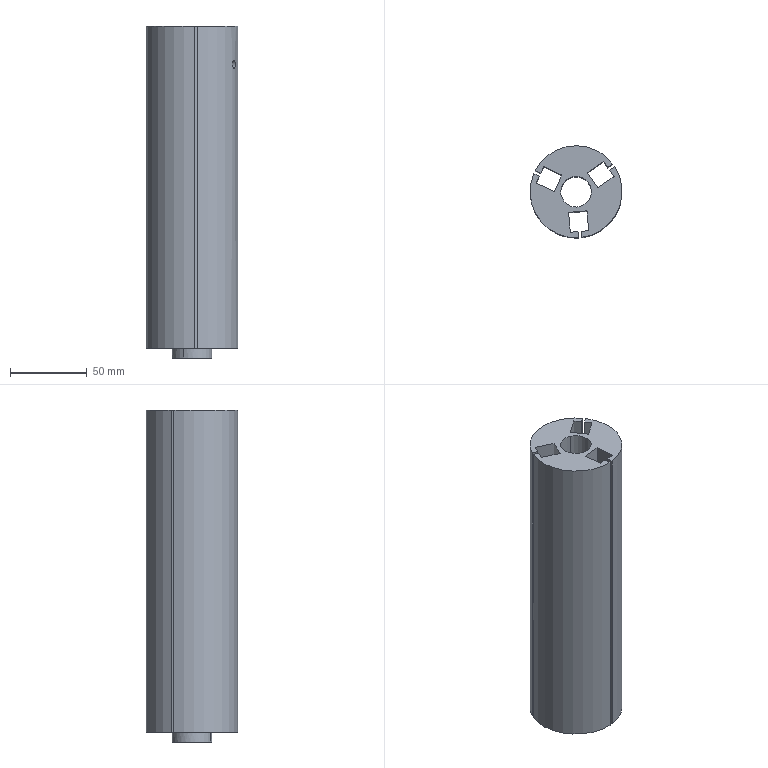Component | SolidWorks | JYTBJ-HeaderPlateRotatingAxisBarrel-1 | 1 solid | 48 faces | box 60 x 60 x 216.5 mm | volume 423997 mm3 | plane 26 | cylinder 16 | cone 6 | commonest cylinder face diameters 6 x6 60 x4 5 x2 20 x2 26 x2
build123d program:
from build123d import *

# Parameters (mm, degrees)
SKETCH1_R             = 30
BOSS_EXTRUDE1_DEPTH   = 210
SKETCH2_R             = 13
BOSS_EXTRUDE2_DEPTH   = 6.5
SKETCH3_R             = 10
CUT_EXTRUDE1_DEPTH    = 221.618
CUT_EXTRUDE2_DEPTH    = 215.243
CIRPATTERN1_COUNT     = 3
CIRPATTERN2_COUNT     = 3
M6_TAPPED_HOLE1_D     = 5
M6_TAPPED_HOLE1_DEPTH = 30
M6_TAPPED_HOLE1_TIP   = 1.502


with BuildPart() as part:
    # Sketch1 → Boss-Extrude1 (new body)
    with BuildSketch(Plane.XY):
        Circle(SKETCH1_R)
    extrude(amount=BOSS_EXTRUDE1_DEPTH)

    # Sketch2 → Boss-Extrude2 (add)
    with BuildSketch(Plane.XY.offset(210)):
        with Locations(Location((0, 0, 0), (0, 0, 180))):
            Circle(SKETCH2_R)
    extrude(amount=BOSS_EXTRUDE2_DEPTH)

    # Sketch3 → Cut-Extrude1 (cut, through all)
    with BuildSketch(Plane.XY.offset(216.5)):
        Circle(SKETCH3_R)
    extrude(amount=-CUT_EXTRUDE1_DEPTH, mode=Mode.SUBTRACT)

    # Sketch4 → Cut-Extrude2 (cut, through all)
    with BuildSketch(Plane.XY.offset(210)):
        Polygon((1, 26), (6, 26), (6, 13), (-6, 13), (-6, 26), (-1, 26), (-1, 36.22), (1, 36.22), align=None)
    cut_extrude2 = extrude(amount=-CUT_EXTRUDE2_DEPTH, mode=Mode.SUBTRACT)

    # CirPattern1: Cut-Extrude2 ×3 about axis
    cirpattern1_axis = Axis((0, 0, 0), (0, 0, 1))
    for i in range(1, CIRPATTERN1_COUNT):
        add(cut_extrude2.rotate(cirpattern1_axis, i * 360 / CIRPATTERN1_COUNT), mode=Mode.SUBTRACT)

    # Sketch5 → M6 Tapped Hole2 (revolve, cut)
    with BuildSketch(Plane(origin=(0, -20, 210), x_dir=(0, -1, 0), z_dir=(1, 0, 0))):
        Polygon((0, 0), (0, 18.803), (3, 17), (3, 0), align=None)
    m6_tapped_hole2 = revolve(axis=Axis((0, -20, 216.35), (0, 0, -1)), mode=Mode.SUBTRACT)

    # CirPattern2: M6 Tapped Hole2 ×3 about axis
    cirpattern2_axis = Axis((0, 0, 0), (0, 0, 1))
    for i in range(1, CIRPATTERN2_COUNT):
        add(m6_tapped_hole2.rotate(cirpattern2_axis, i * 360 / CIRPATTERN2_COUNT), mode=Mode.SUBTRACT)

    # M6 Tapped Hole1
    with Locations(Plane(origin=(0, -30, 25), x_dir=(-1, 0, 0), z_dir=(0, -1, 0))):
        with Locations((0, 0)):
            Hole(M6_TAPPED_HOLE1_D / 2, depth=M6_TAPPED_HOLE1_DEPTH)
            with Locations((0, 0, -(M6_TAPPED_HOLE1_DEPTH + M6_TAPPED_HOLE1_TIP / 2))):  # 118° drill point
                Cone(0, M6_TAPPED_HOLE1_D / 2, M6_TAPPED_HOLE1_TIP, mode=Mode.SUBTRACT)


solid = part.part

# Placed as in the assembly
solid = solid.moved(Location((3.373, 96.878, 258.5), (180, 0, 115.119)))